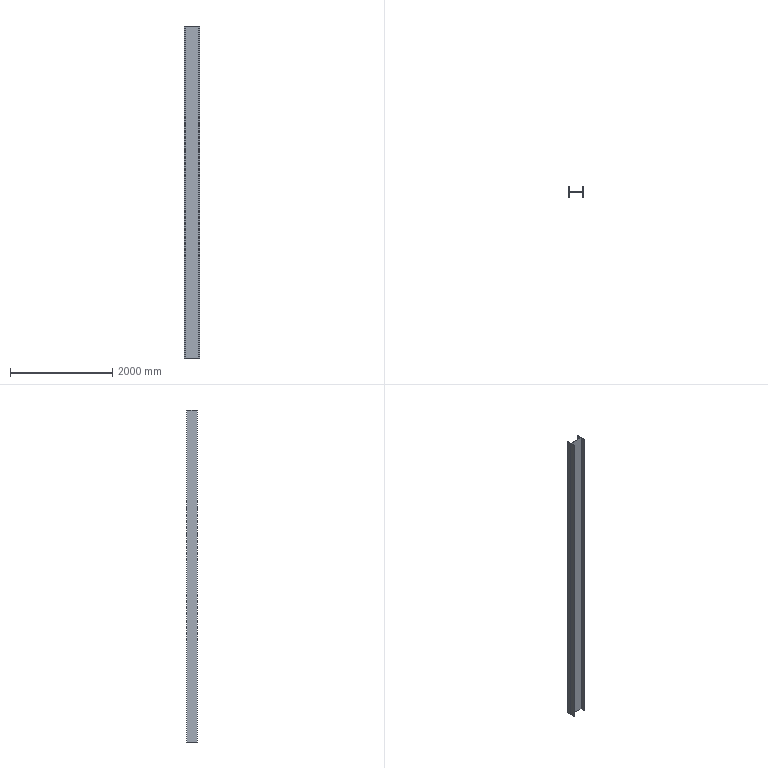Component | NX | 59_11 | 1 solid | 14 faces | volume 45240000 mm3 | plane 14